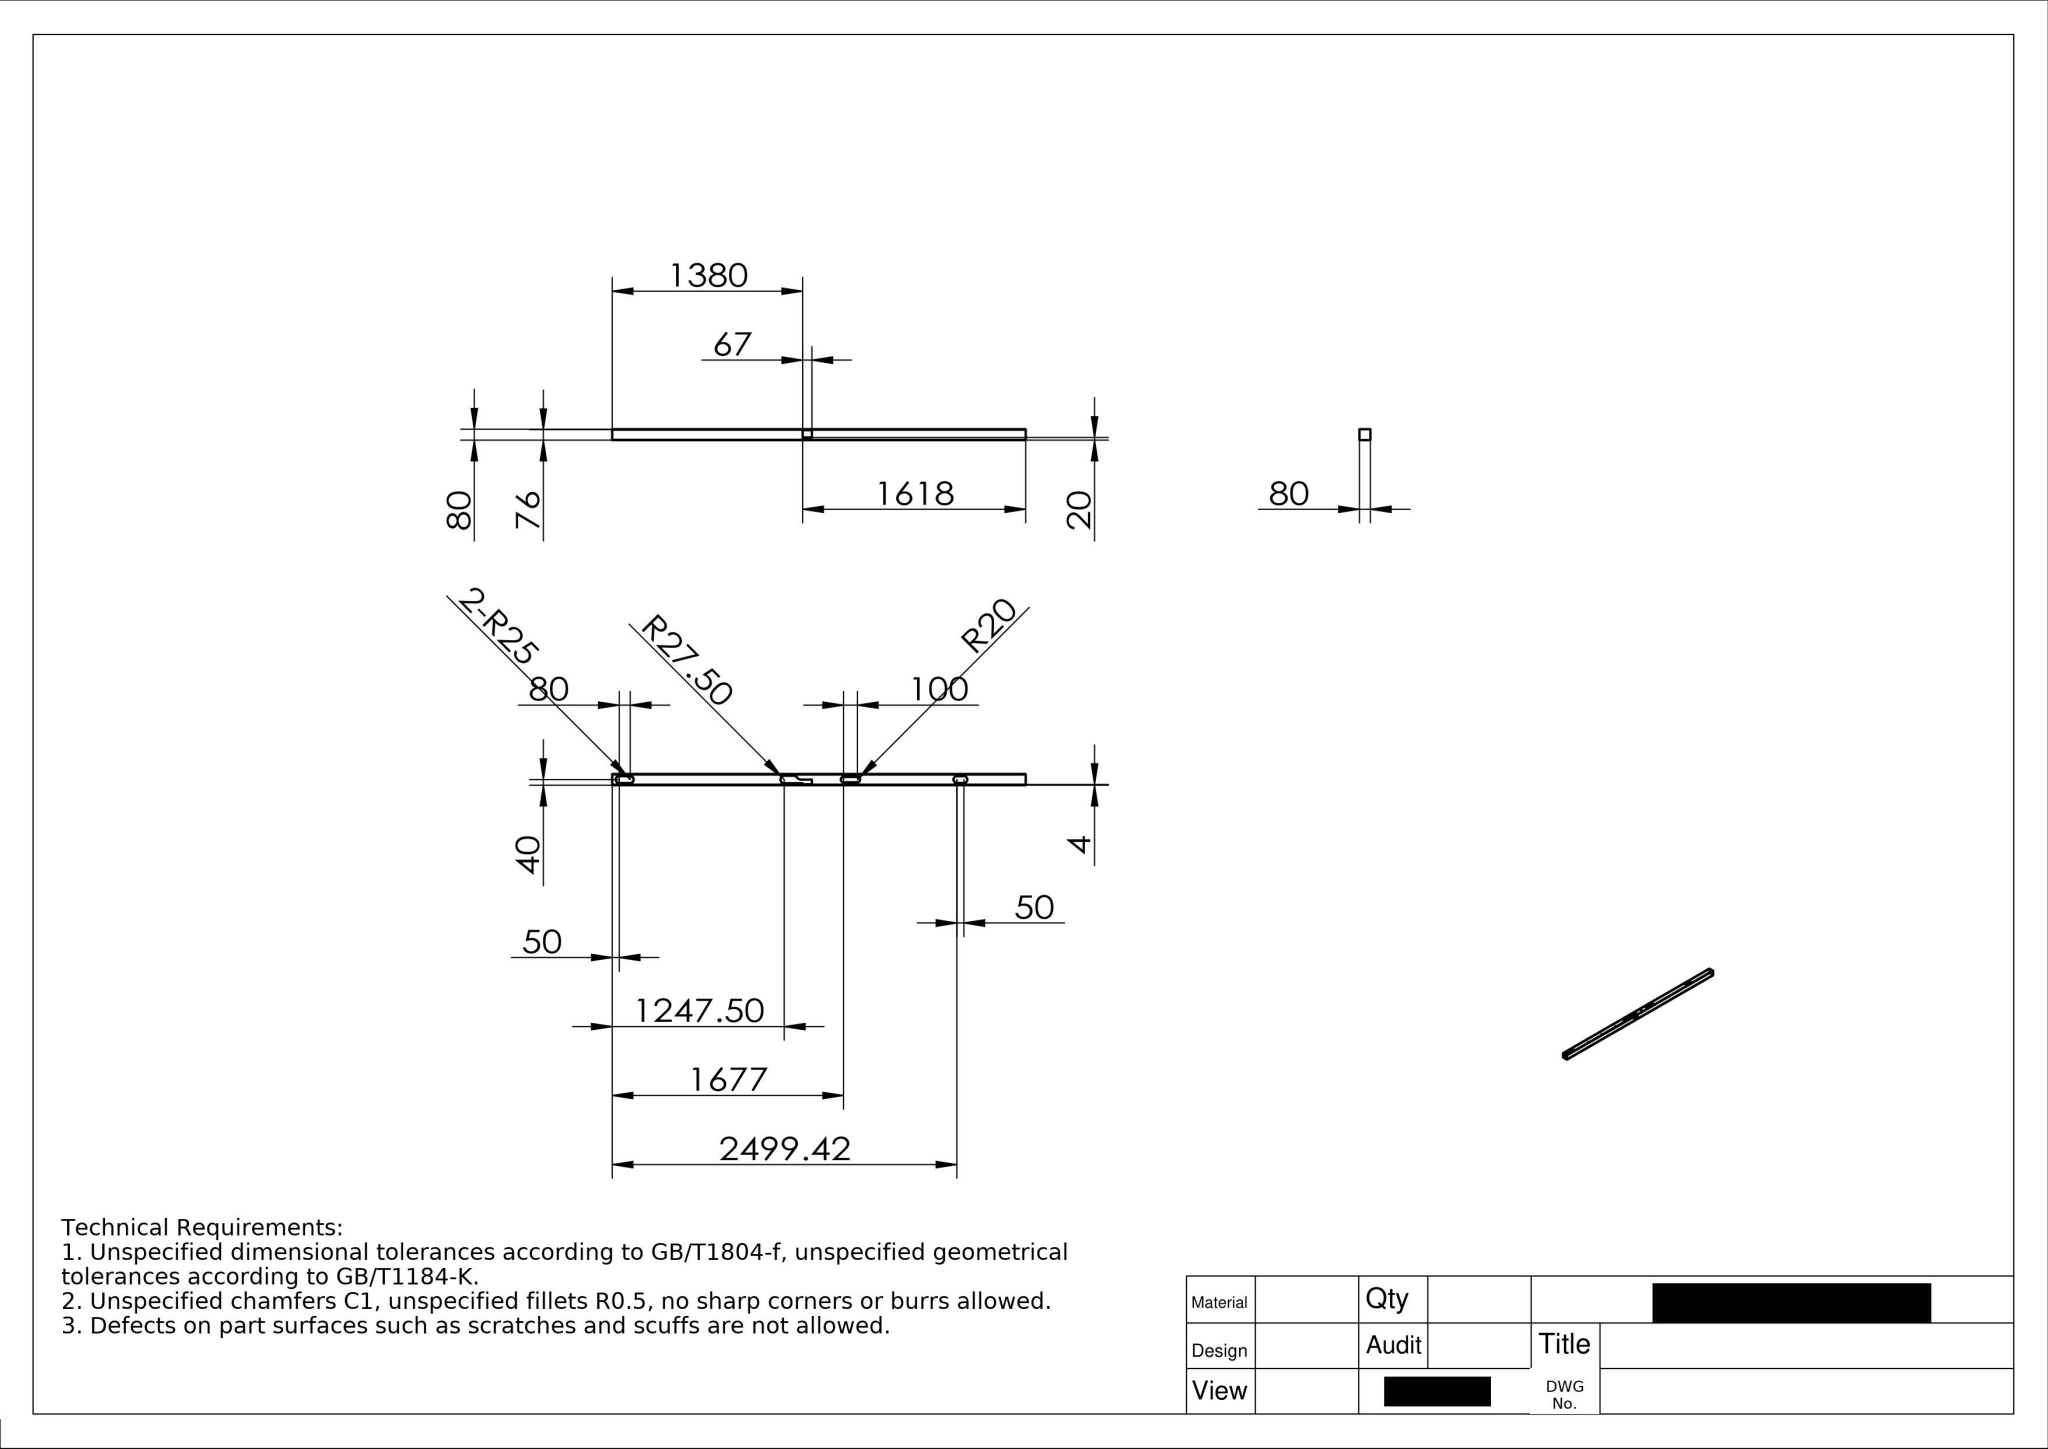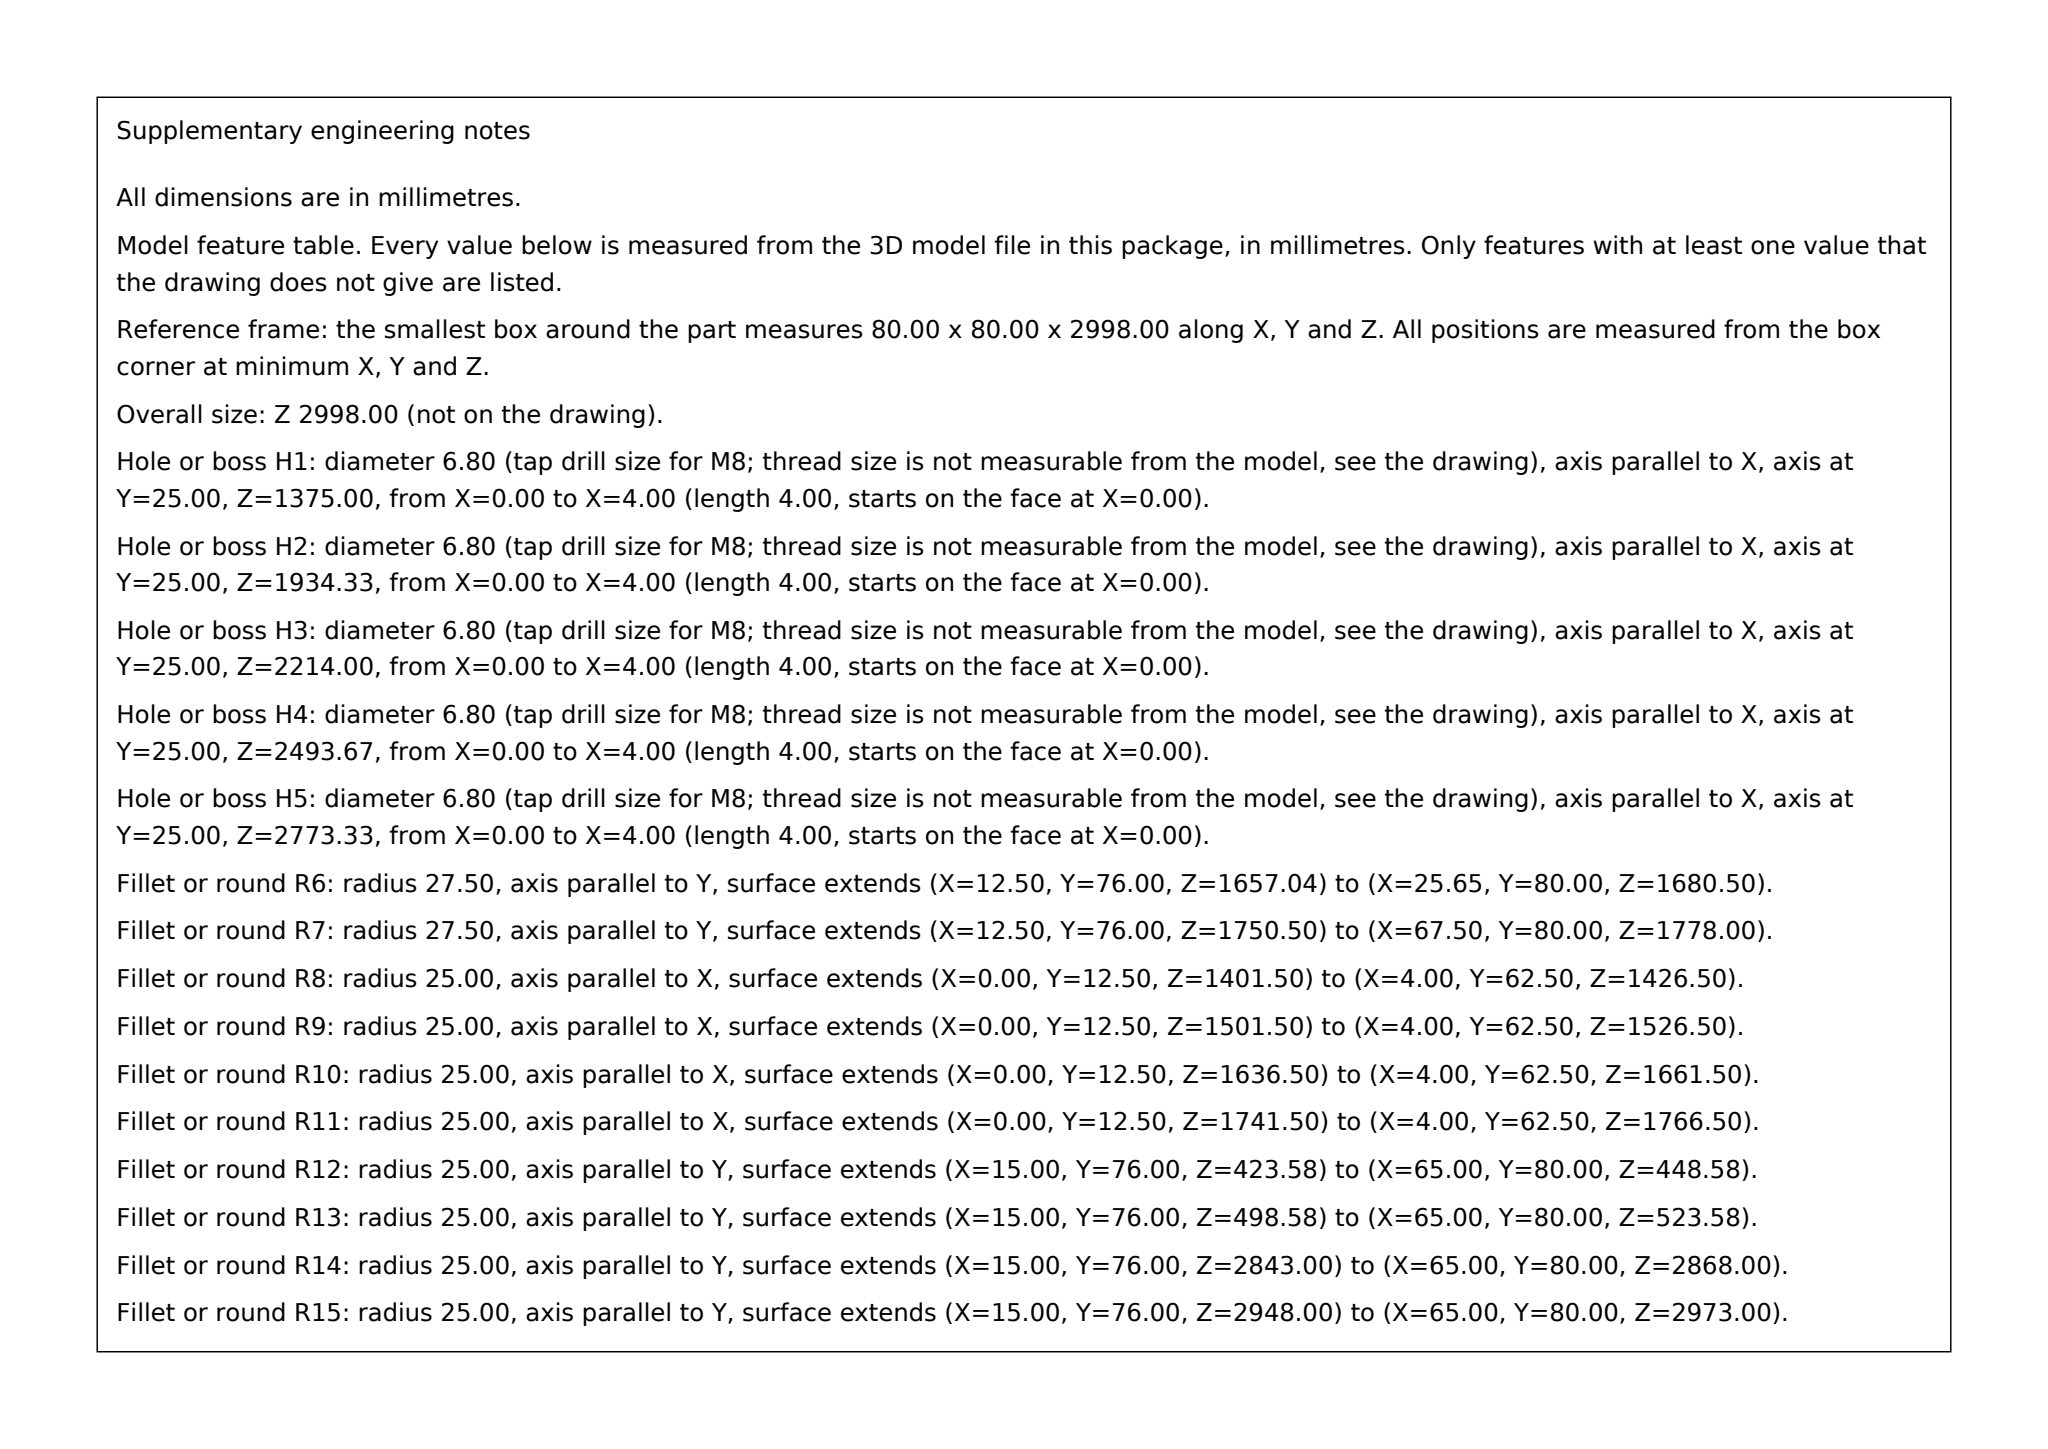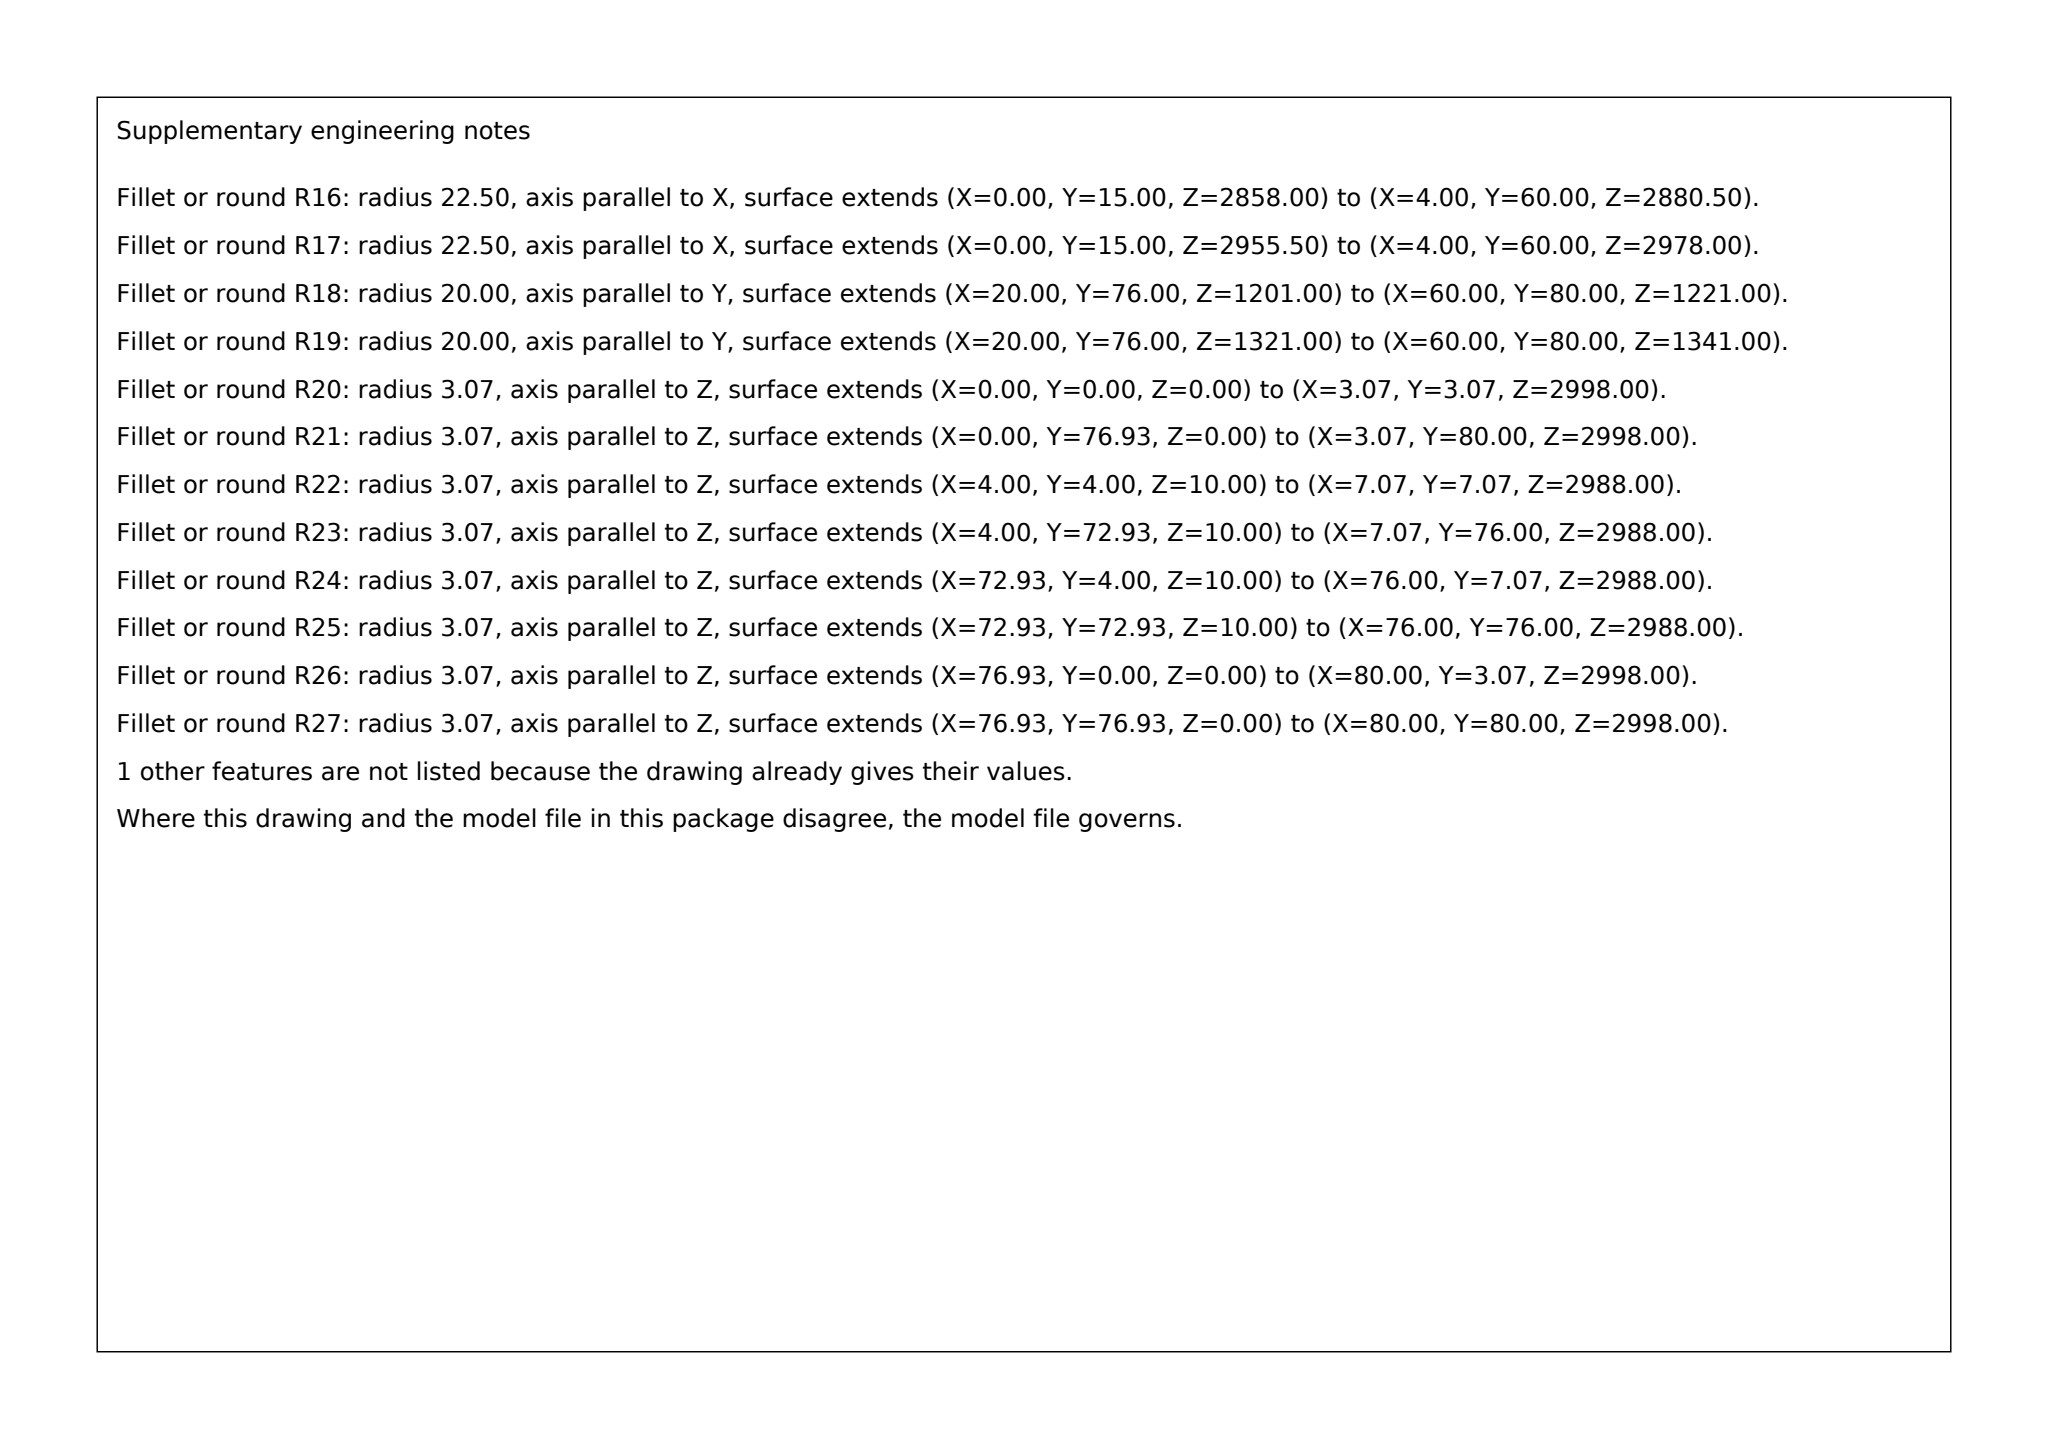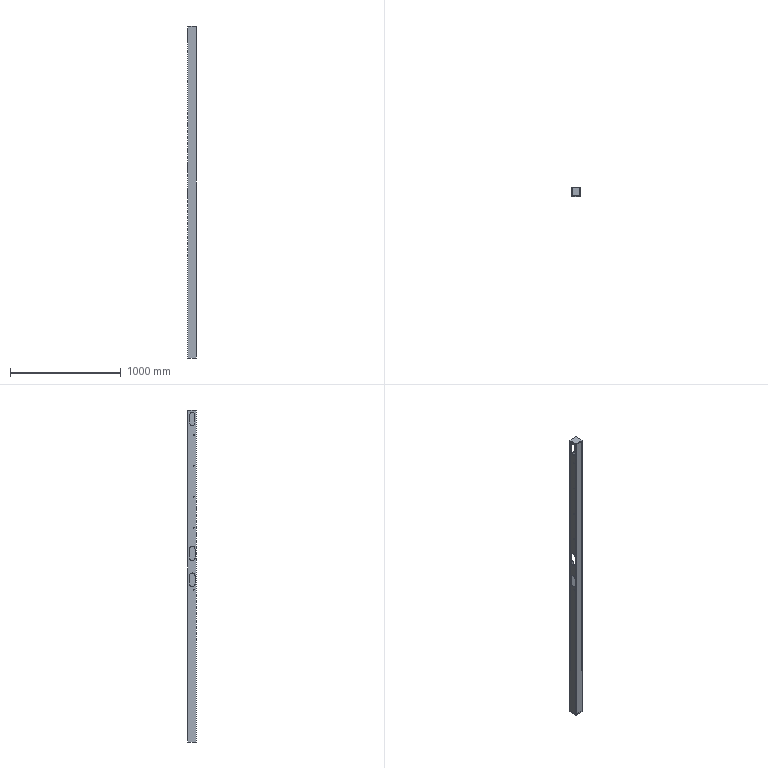Part | SolidWorks | mm | 1 solid | 72 faces | box 80 x 80 x 2998 mm | volume 3563651 mm3 | cylinder 42 | plane 30 | commonest cylinder face diameters 50 x12 6.8 x10 6.148 x10 45 x3 40 x3 55 x3 60 x1
build123d program:
from build123d import *

# Parameters (mm, degrees)
BASE_EXTRUDE_DEPTH    = 2998
SKETCH2_W             = 78.199
SKETCH2_H             = 78.199
BOSS_EXTRUDE1_DEPTH   = 10
SKETCH3_W             = 78.199
SKETCH3_H             = 78.199
BOSS_EXTRUDE2_DEPTH   = 10
CUT_EXTRUDE4_DEPTH    = 10
CUT_EXTRUDE9_DEPTH    = 60
M8_TAPPED_HOLE1_D     = 6.8
M8_TAPPED_HOLE1_DEPTH = 19.75
M8_TAPPED_HOLE1_TIP   = 2.043
CUT_EXTRUDE12_DEPTH   = 10
FILLET2_R             = 30
CUT_EXTRUDE15_DEPTH   = 10
CUT_EXTRUDE16_DEPTH   = 10
CUT_EXTRUDE17_DEPTH   = 10
CUT_EXTRUDE18_DEPTH   = 10


with BuildPart() as part:
    # Sketch1 → Base-Extrude (new body)
    with BuildSketch(Plane.XY):
        with BuildLine():
            Line((-36.926, 40), (36.926, 40))
            ThreePointArc((36.926, 40), (39.1, 39.1), (40, 36.926))
            Line((40, 36.926), (40, -36.926))
            ThreePointArc((40, -36.926), (39.1, -39.1), (36.926, -40))
            Line((36.926, -40), (-36.926, -40))
            ThreePointArc((-36.926, -40), (-39.1, -39.1), (-40, -36.926))
            Line((-40, -36.926), (-40, 36.926))
            ThreePointArc((-40, 36.926), (-39.1, 39.1), (-36.926, 40))
        make_face()
        with BuildLine():
            Line((-32.926, 36), (32.926, 36))
            ThreePointArc((32.926, 36), (35.1, 35.1), (36, 32.926))
            Line((36, 32.926), (36, -32.926))
            ThreePointArc((36, -32.926), (35.1, -35.1), (32.926, -36))
            Line((32.926, -36), (-32.926, -36))
            ThreePointArc((-32.926, -36), (-35.1, -35.1), (-36, -32.926))
            Line((-36, -32.926), (-36, 32.926))
            ThreePointArc((-36, 32.926), (-35.1, 35.1), (-32.926, 36))
        make_face(mode=Mode.SUBTRACT)
    extrude(amount=BASE_EXTRUDE_DEPTH)

    # Sketch2 → Boss-Extrude1 (add)
    with BuildSketch(Plane.XY.offset(2998)):
        Rectangle(SKETCH2_W, SKETCH2_H)
    extrude(amount=-BOSS_EXTRUDE1_DEPTH)

    # Sketch3 → Boss-Extrude2 (add)
    with BuildSketch(Plane(origin=(0, 0, 0), x_dir=(-1, 0, 0), z_dir=(0, 0, -1))):
        Rectangle(SKETCH3_W, SKETCH3_H)
    extrude(amount=-BOSS_EXTRUDE2_DEPTH)

    # Sketch11 → Cut-Extrude4 (cut)
    with BuildSketch(Plane(origin=(0, 40, 0), x_dir=(1, 0, 0), z_dir=(0, 1, 0))):
        with BuildLine():
            Line((-27.5, -1750.5), (-27.5, -1680.5))
            ThreePointArc((-27.5, -1680.5), (0, -1653), (27.5, -1680.5))
            Line((27.5, -1680.5), (27.5, -1750.5))
            ThreePointArc((27.5, -1750.5), (0, -1778), (-27.5, -1750.5))
        make_face()
    extrude(amount=-CUT_EXTRUDE4_DEPTH, mode=Mode.SUBTRACT)

    # Sketch13 → Cut-Extrude9 (cut)
    with BuildSketch(Plane(origin=(0, 40, 0), x_dir=(1, 0, 0), z_dir=(0, 1, 0))):
        with BuildLine():
            Line((0, -1653), (0, -1551))
            Line((0, -1551), (50, -1551))
            Line((50, -1551), (50, -1618))
            Line((50, -1618), (27.5, -1618))
            Line((27.5, -1618), (27.5, -1680.5))
            ThreePointArc((27.5, -1680.5), (19.445, -1661.055), (0, -1653))
        make_face()
    extrude(amount=-CUT_EXTRUDE9_DEPTH, mode=Mode.SUBTRACT)

    # M8 Tapped Hole1
    with Locations(Plane.ZY.offset(40)):
        with Locations((2773.333, -15), (2493.667, -15), (2214, -15), (1934.333, -15), (1375, -15)):
            Hole(M8_TAPPED_HOLE1_D / 2, depth=M8_TAPPED_HOLE1_DEPTH)
            with Locations((0, 0, -(M8_TAPPED_HOLE1_DEPTH + M8_TAPPED_HOLE1_TIP / 2))):  # 118° drill point
                Cone(0, M8_TAPPED_HOLE1_D / 2, M8_TAPPED_HOLE1_TIP, mode=Mode.SUBTRACT)

    # Sketch18 → Cut-Extrude12 (cut)
    with BuildSketch(Plane(origin=(0, 40, 0), x_dir=(1, 0, 0), z_dir=(0, 1, 0))):
        with BuildLine():
            Line((-25, -2948), (-25, -2868))
            ThreePointArc((-25, -2868), (0, -2843), (25, -2868))
            Line((25, -2868), (25, -2948))
            ThreePointArc((25, -2948), (0, -2973), (-25, -2948))
        make_face()
    extrude(amount=-CUT_EXTRUDE12_DEPTH, mode=Mode.SUBTRACT)

    # Fillet2
    fillet2_edges = [part.edges().sort_by_distance(p)[0] for p in [
        (0, 38, 1653),
    ]]
    fillet(fillet2_edges, radius=FILLET2_R)

    # Sketch22 → Cut-Extrude15 (cut)
    with BuildSketch(Plane(origin=(0, 40, 0), x_dir=(1, 0, 0), z_dir=(0, 1, 0))):
        with BuildLine():
            Line((-20, -1321), (-20, -1221))
            ThreePointArc((-20, -1221), (0, -1201), (20, -1221))
            Line((20, -1221), (20, -1321))
            ThreePointArc((20, -1321), (0, -1341), (-20, -1321))
        make_face()
    extrude(amount=-CUT_EXTRUDE15_DEPTH, mode=Mode.SUBTRACT)

    # Sketch23 → Cut-Extrude16 (cut)
    with BuildSketch(Plane.ZY.offset(40)):
        with BuildLine():
            Line((1426.5, 22.5), (1501.5, 22.5))
            ThreePointArc((1501.5, 22.5), (1526.5, -2.5), (1501.5, -27.5))
            Line((1501.5, -27.5), (1426.5, -27.5))
            ThreePointArc((1426.5, -27.5), (1401.5, -2.5), (1426.5, 22.5))
        make_face()
        with BuildLine():
            Line((1661.5, 22.5), (1741.5, 22.5))
            ThreePointArc((1741.5, 22.5), (1766.5, -2.5), (1741.5, -27.5))
            Line((1741.5, -27.5), (1661.5, -27.5))
            ThreePointArc((1661.5, -27.5), (1636.5, -2.5), (1661.5, 22.5))
        make_face()
    extrude(amount=-CUT_EXTRUDE16_DEPTH, mode=Mode.SUBTRACT)

    # Sketch24 → Cut-Extrude17 (cut)
    with BuildSketch(Plane.ZY.offset(40)):
        with BuildLine():
            Line((2880.5, 20), (2955.5, 20))
            ThreePointArc((2955.5, 20), (2978, -2.5), (2955.5, -25))
            Line((2955.5, -25), (2880.5, -25))
            ThreePointArc((2880.5, -25), (2858, -2.5), (2880.5, 20))
        make_face()
    extrude(amount=-CUT_EXTRUDE17_DEPTH, mode=Mode.SUBTRACT)

    # Sketch25 → Cut-Extrude18 (cut)
    with BuildSketch(Plane(origin=(0, 40, 0), x_dir=(1, 0, 0), z_dir=(0, 1, 0))):
        with BuildLine():
            Line((-25, -498.581), (-25, -448.581))
            ThreePointArc((-25, -448.581), (0, -423.581), (25, -448.581))
            Line((25, -448.581), (25, -498.581))
            ThreePointArc((25, -498.581), (0, -523.581), (-25, -498.581))
        make_face()
    extrude(amount=-CUT_EXTRUDE18_DEPTH, mode=Mode.SUBTRACT)


solid = part.part